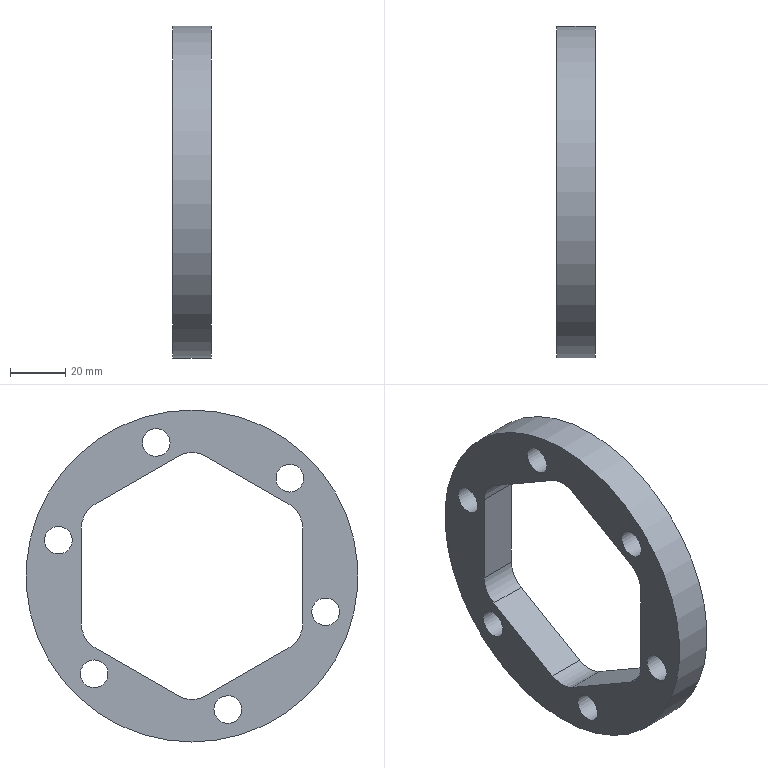Component | NX | TURNTABLE | 1 solid | 21 faces | volume 74595 mm3 | cylinder 13 | plane 8 | commonest cylinder face diameters 10 x6 20 x6 120 x1